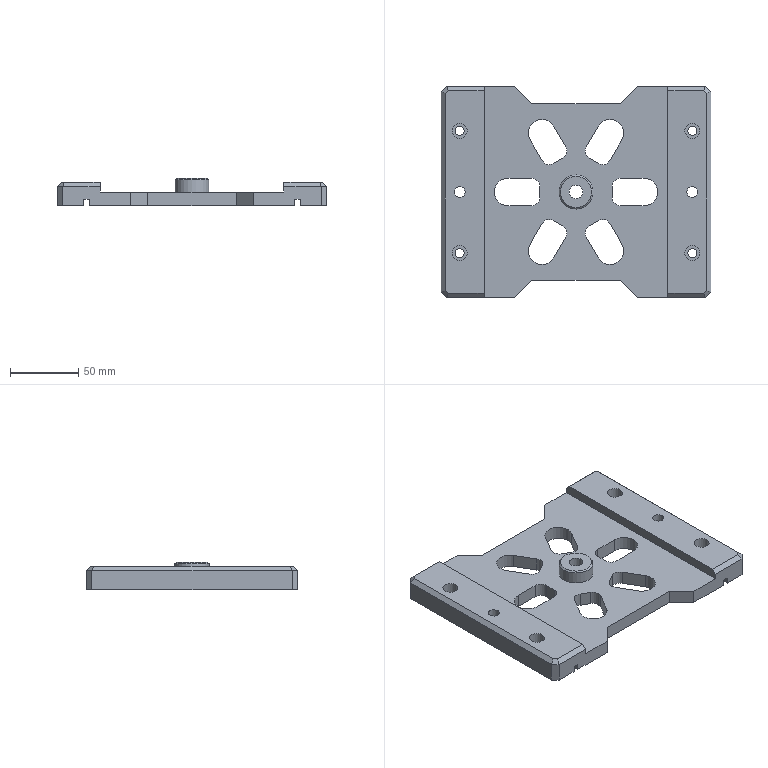Component | NX | TOP_COVER | 1 solid | 94 faces | volume 308000 mm3 | plane 63 | cylinder 30 | cone 1 | commonest cylinder face diameters 12 x12 20 x6 6.6 x4 11 x4 8 x2 25 x1 10 x1